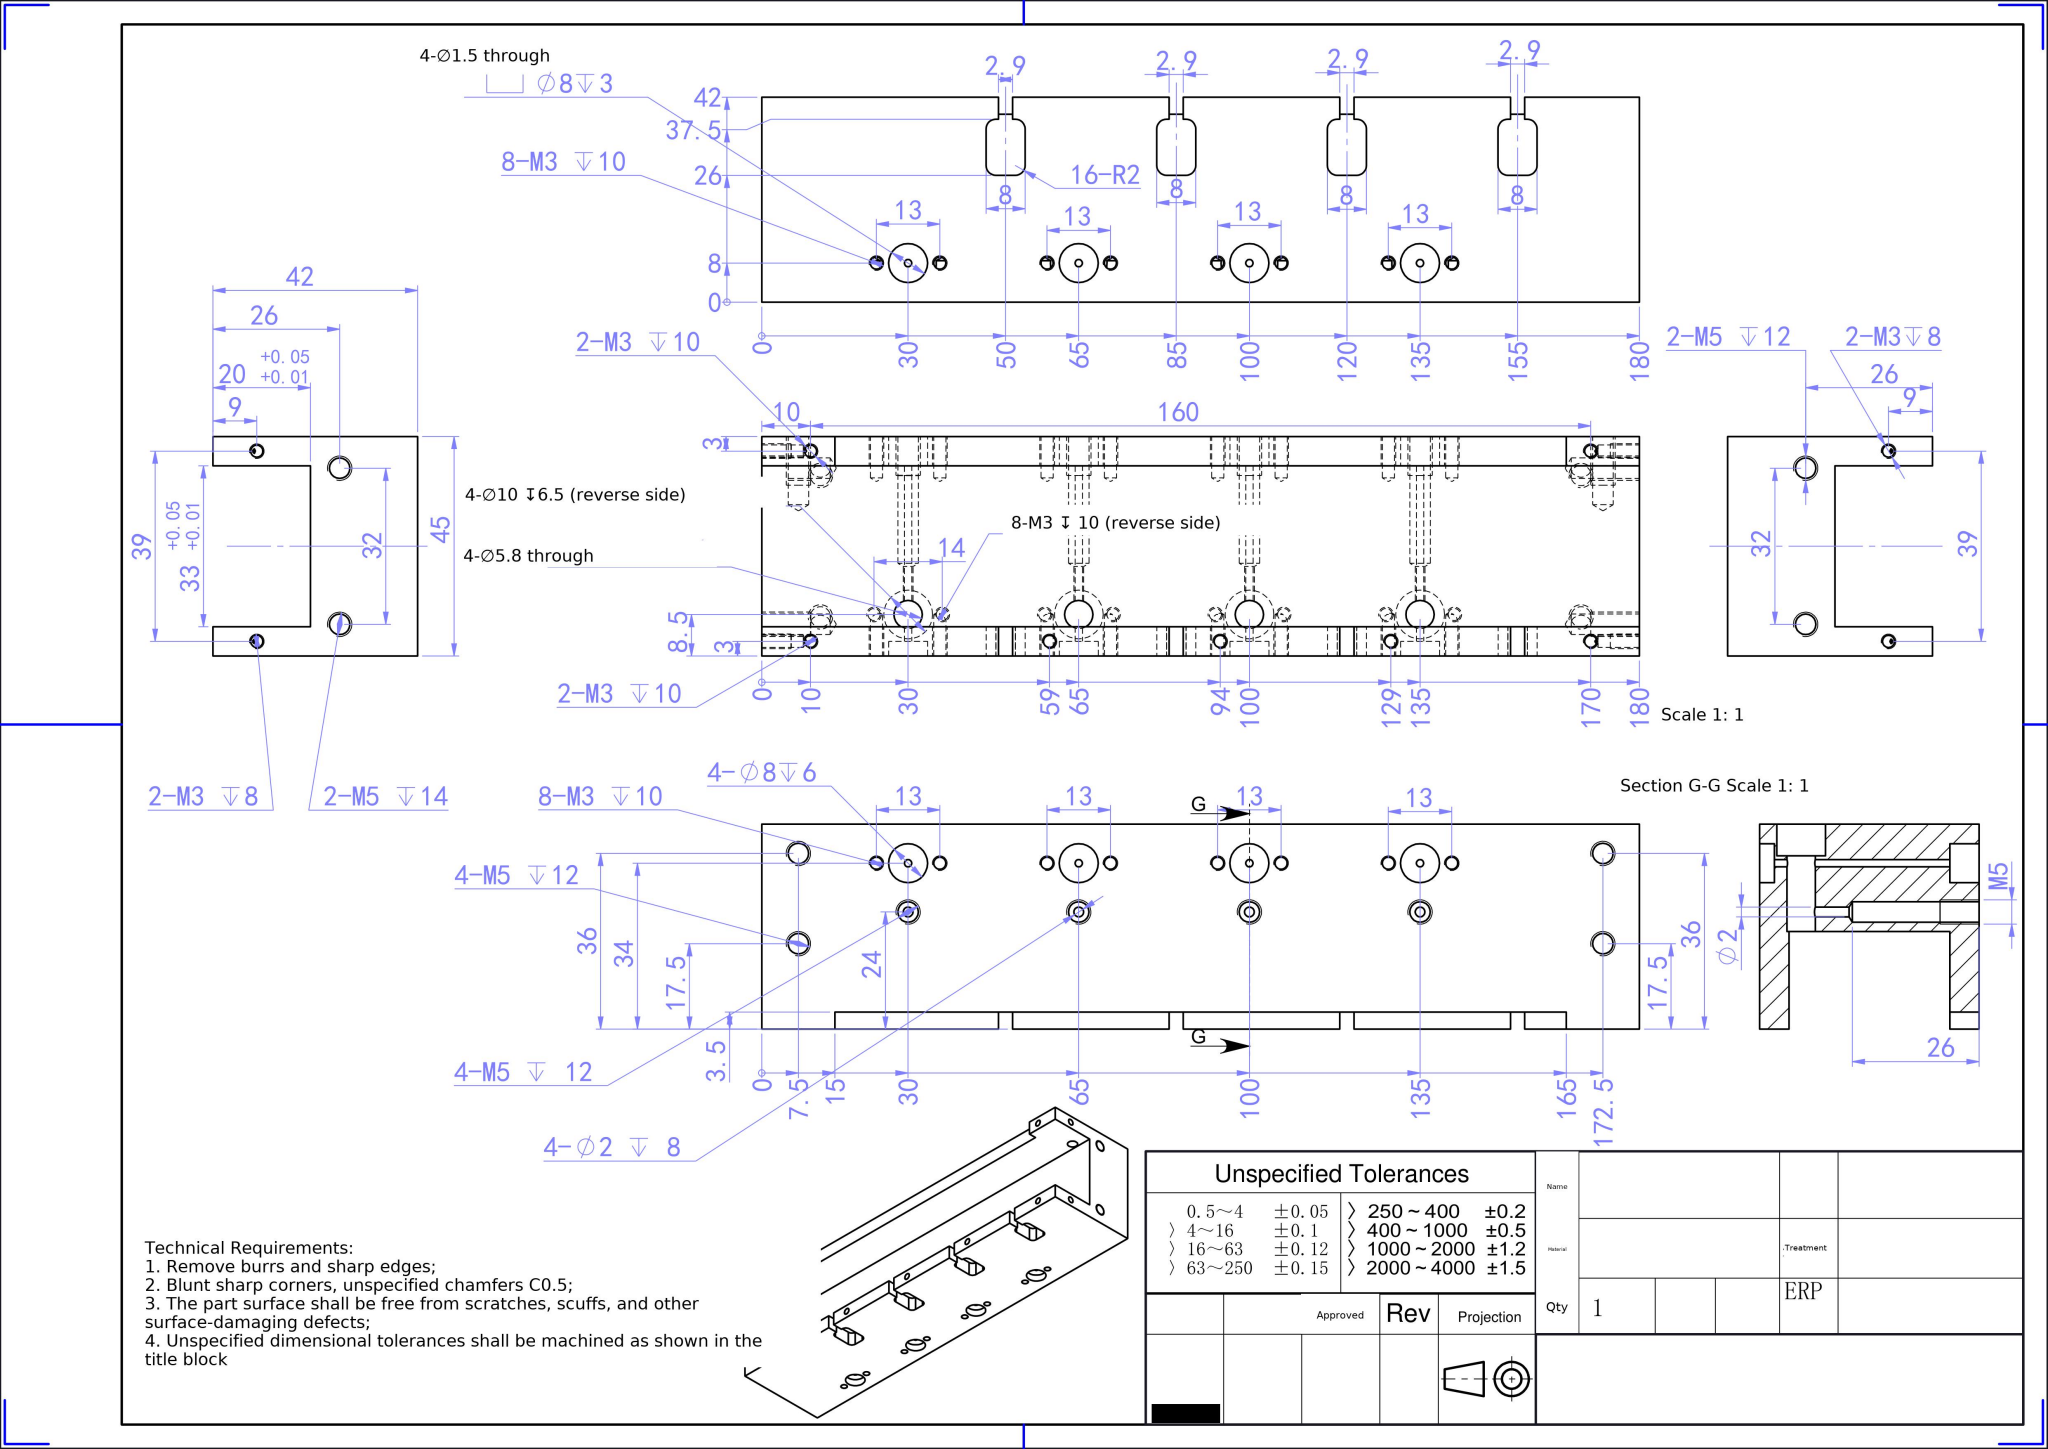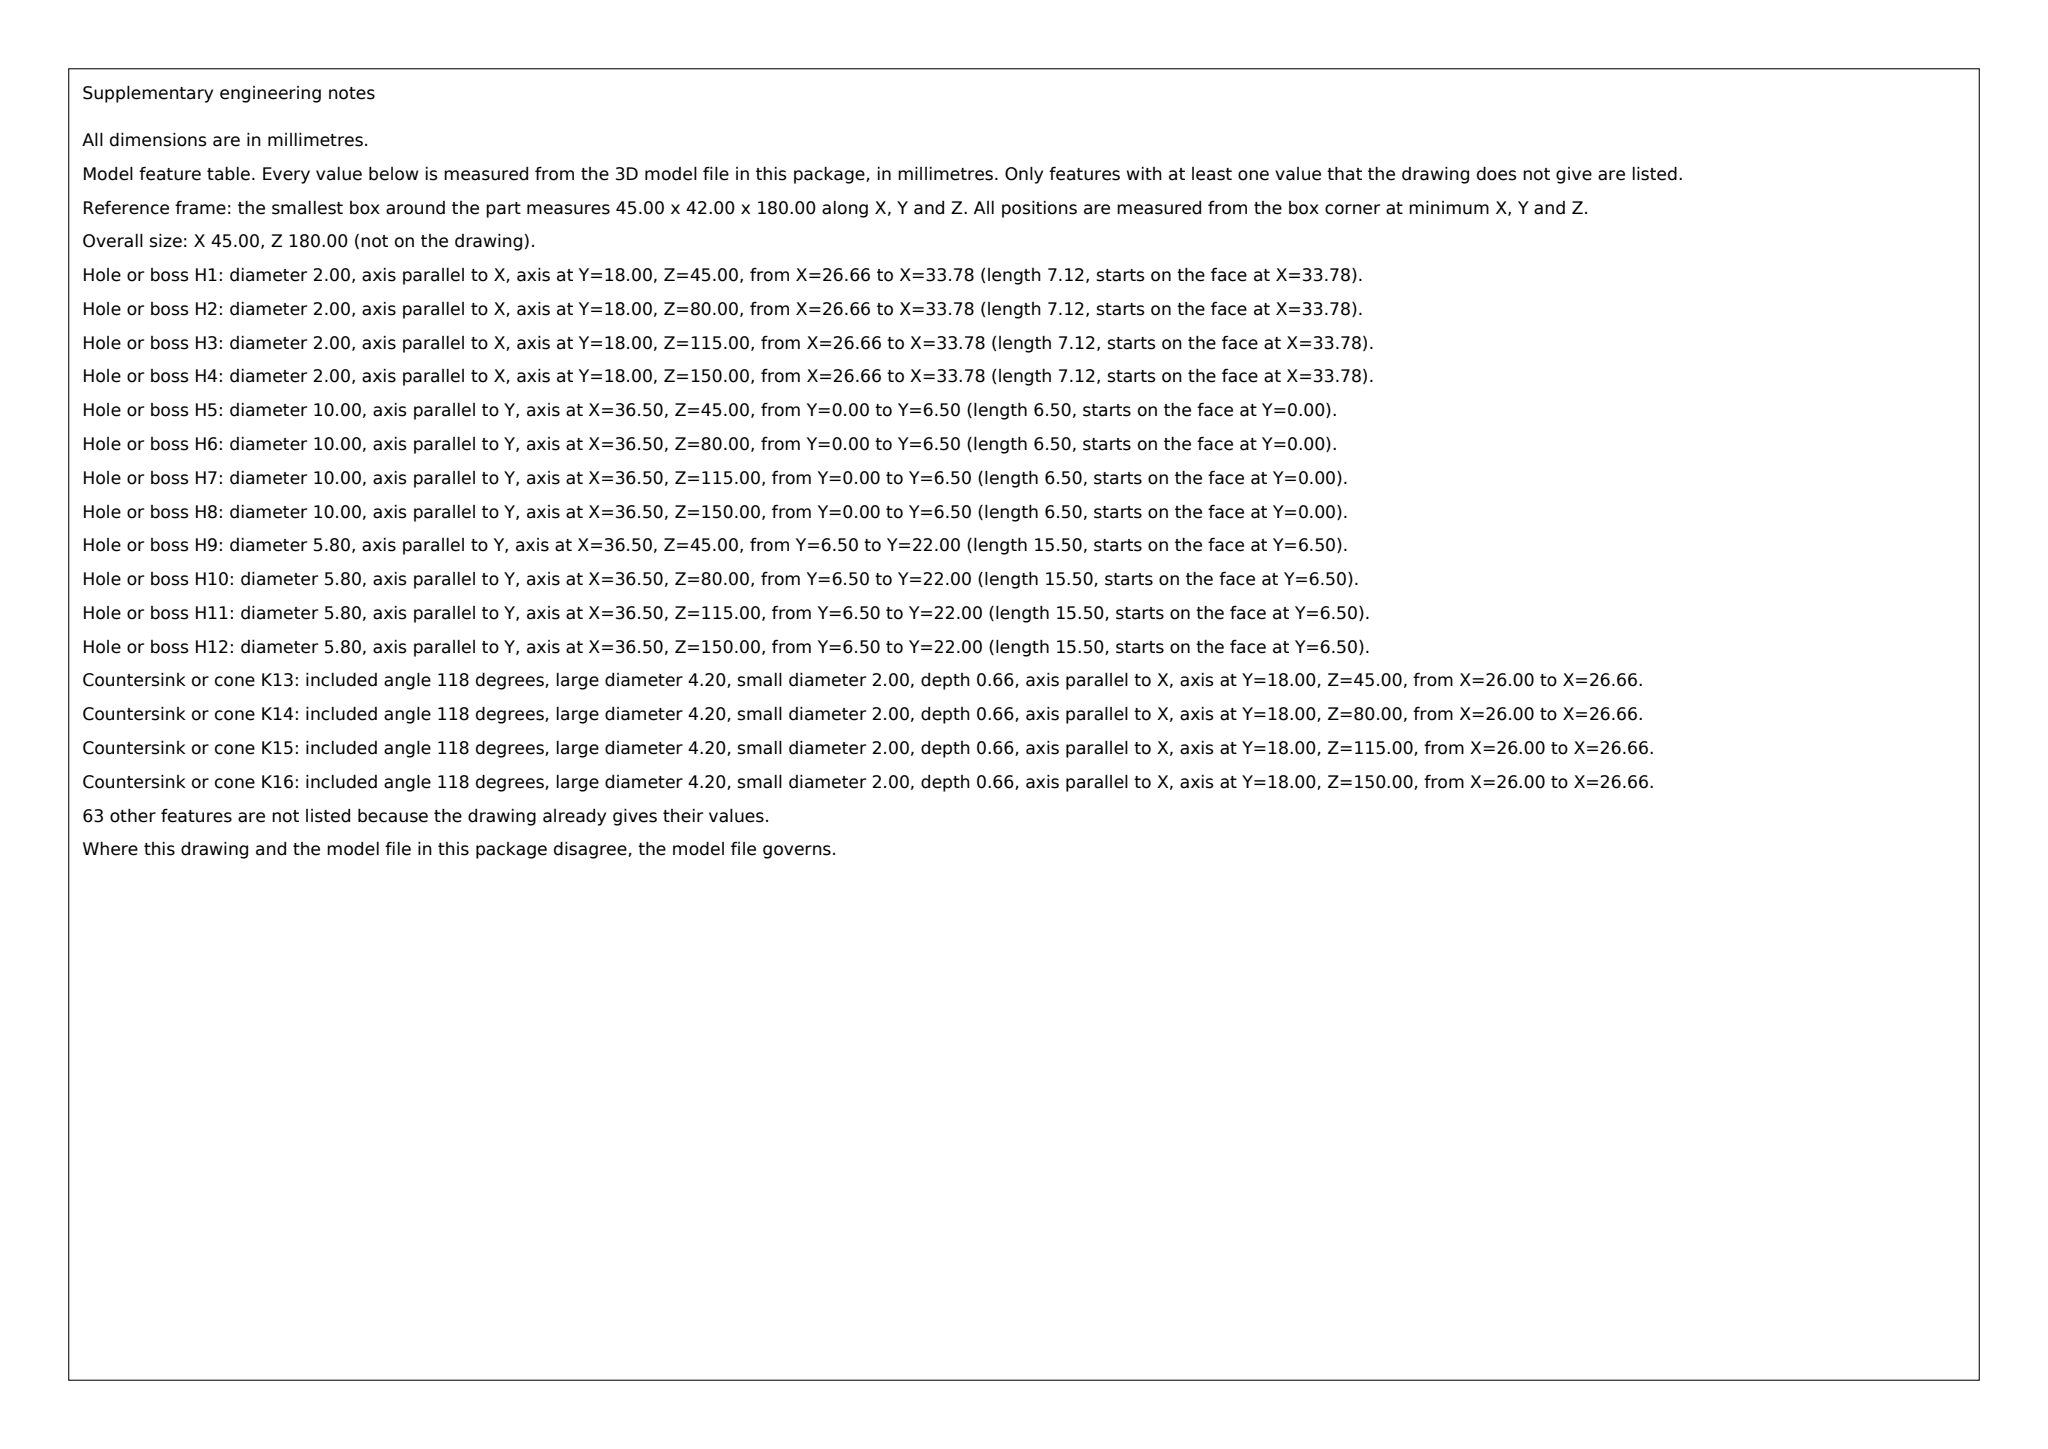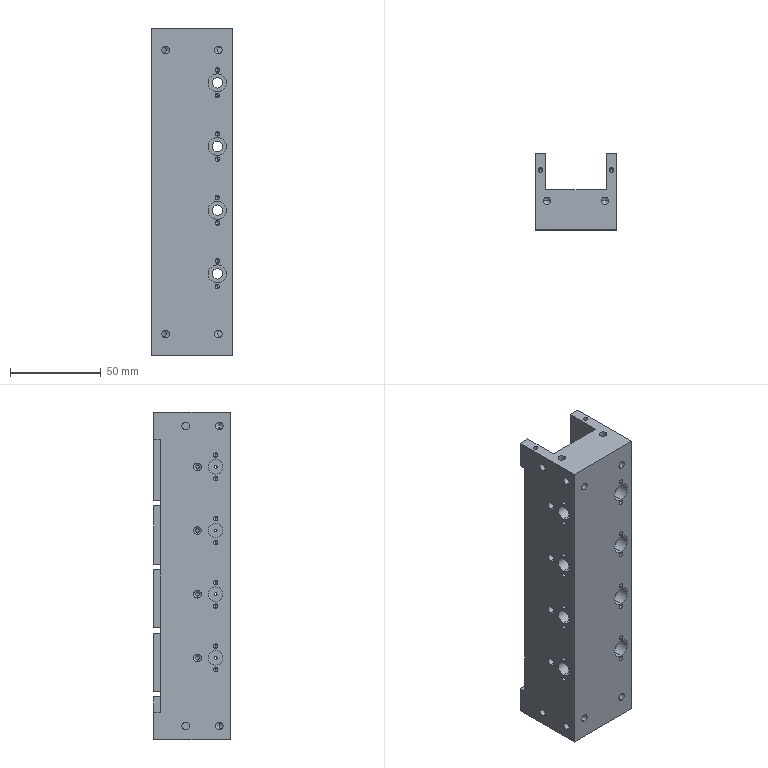Part | SolidWorks | mm | 1 solid | 334 faces | box 45 x 42 x 180 mm | volume 204940 mm3 | cylinder 174 | cone 98 | plane 62 | commonest cylinder face diameters 2.5 x70 4.2 x32 8 x16 1.5 x16 4 x16 2 x8 10 x8 5.8 x8